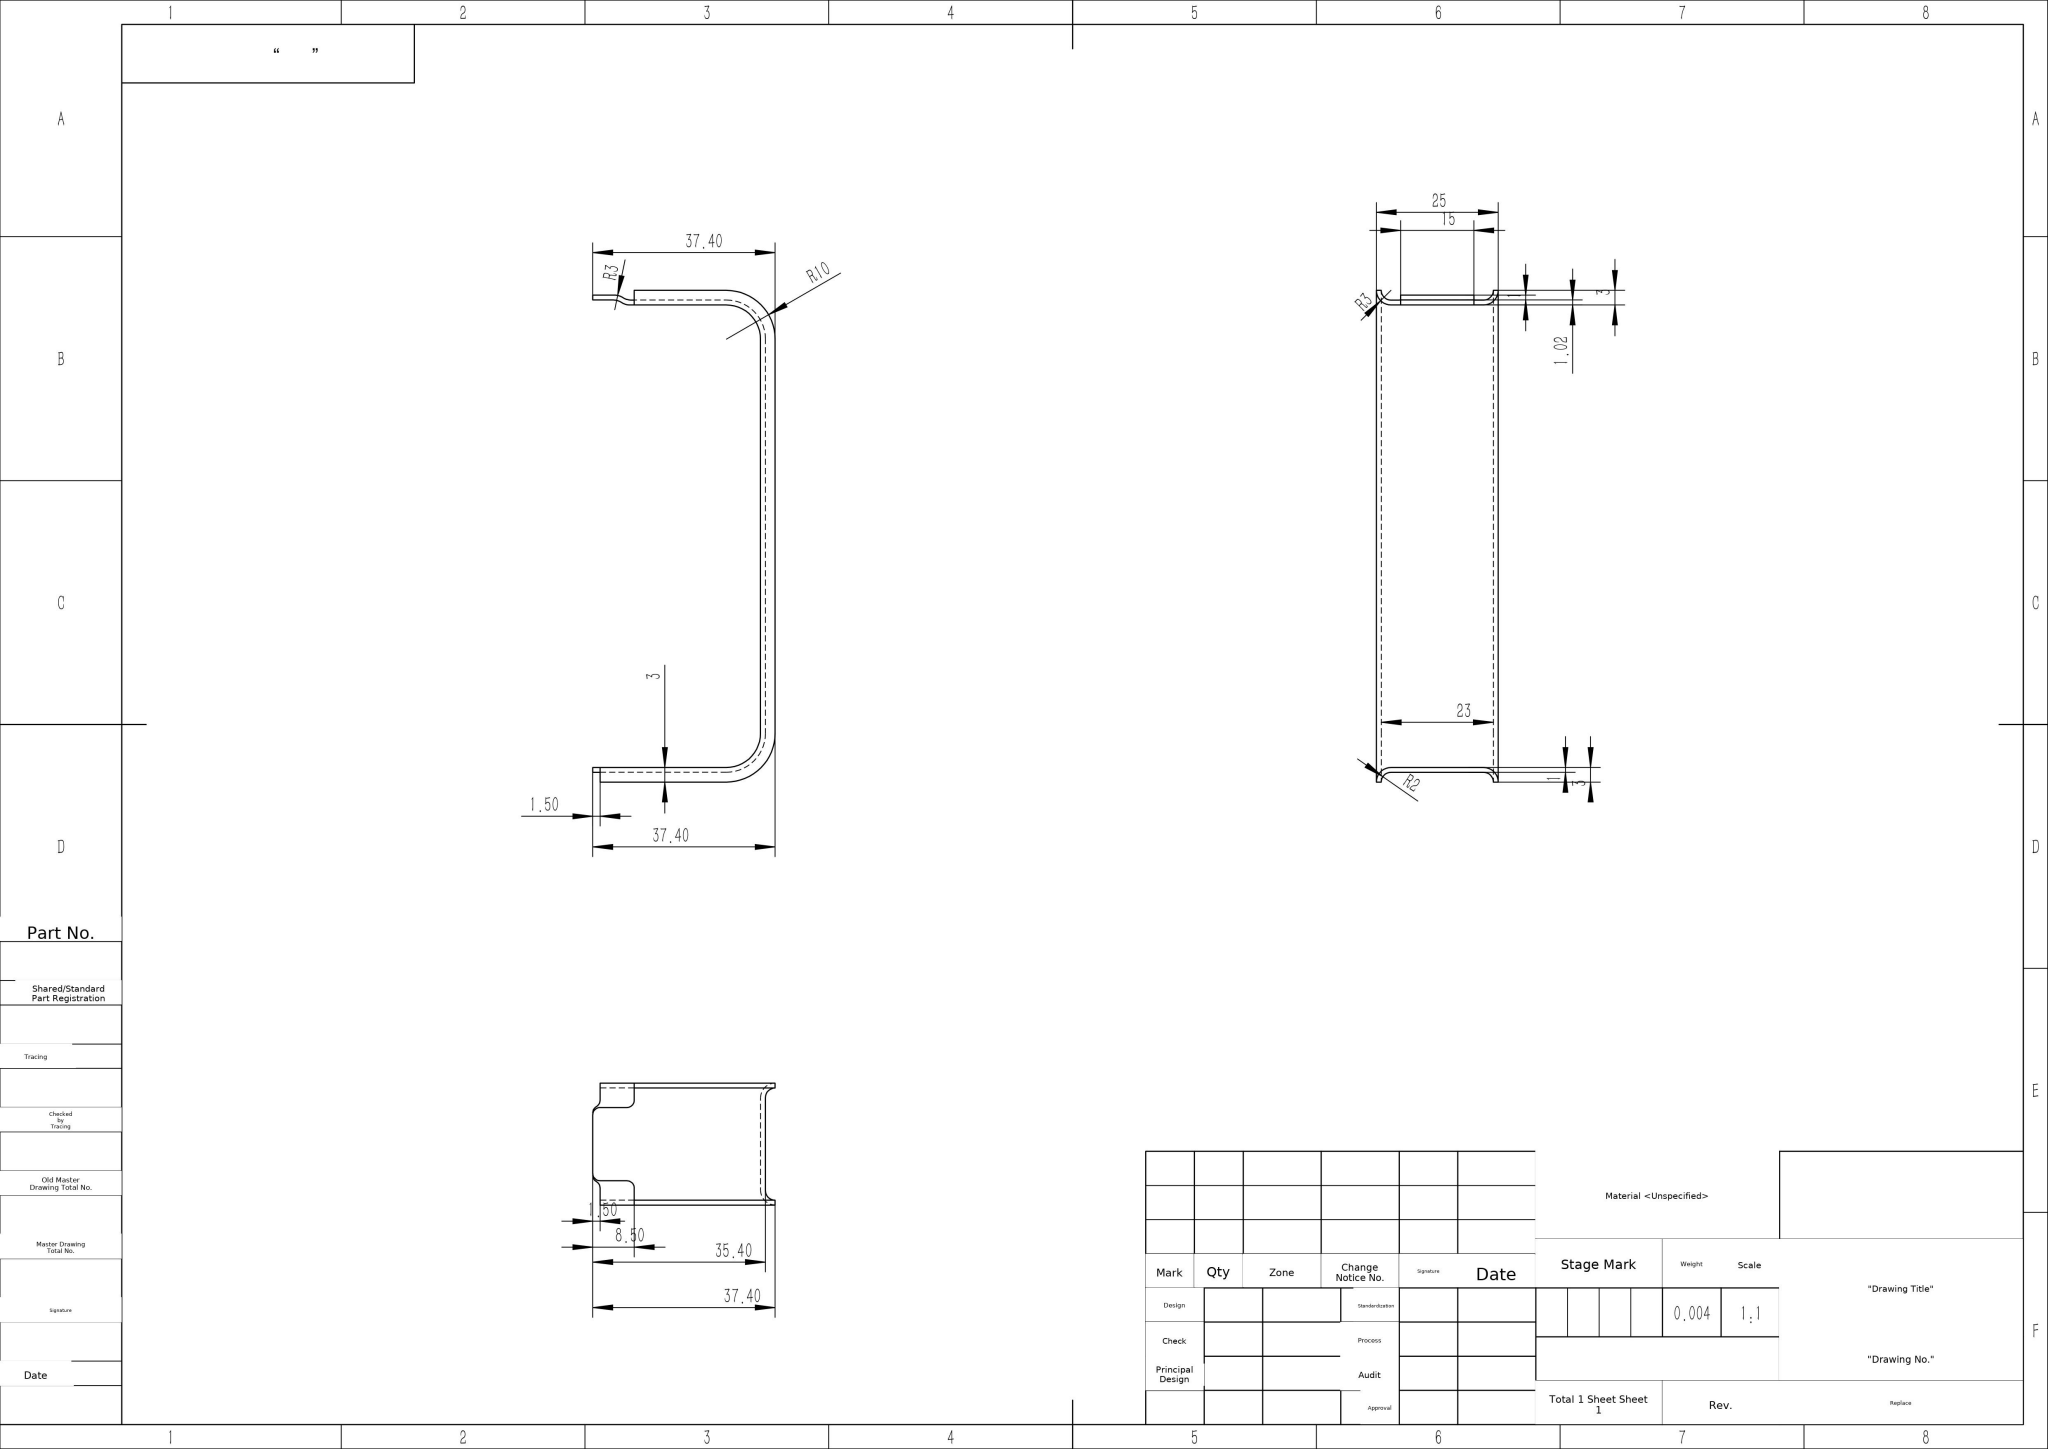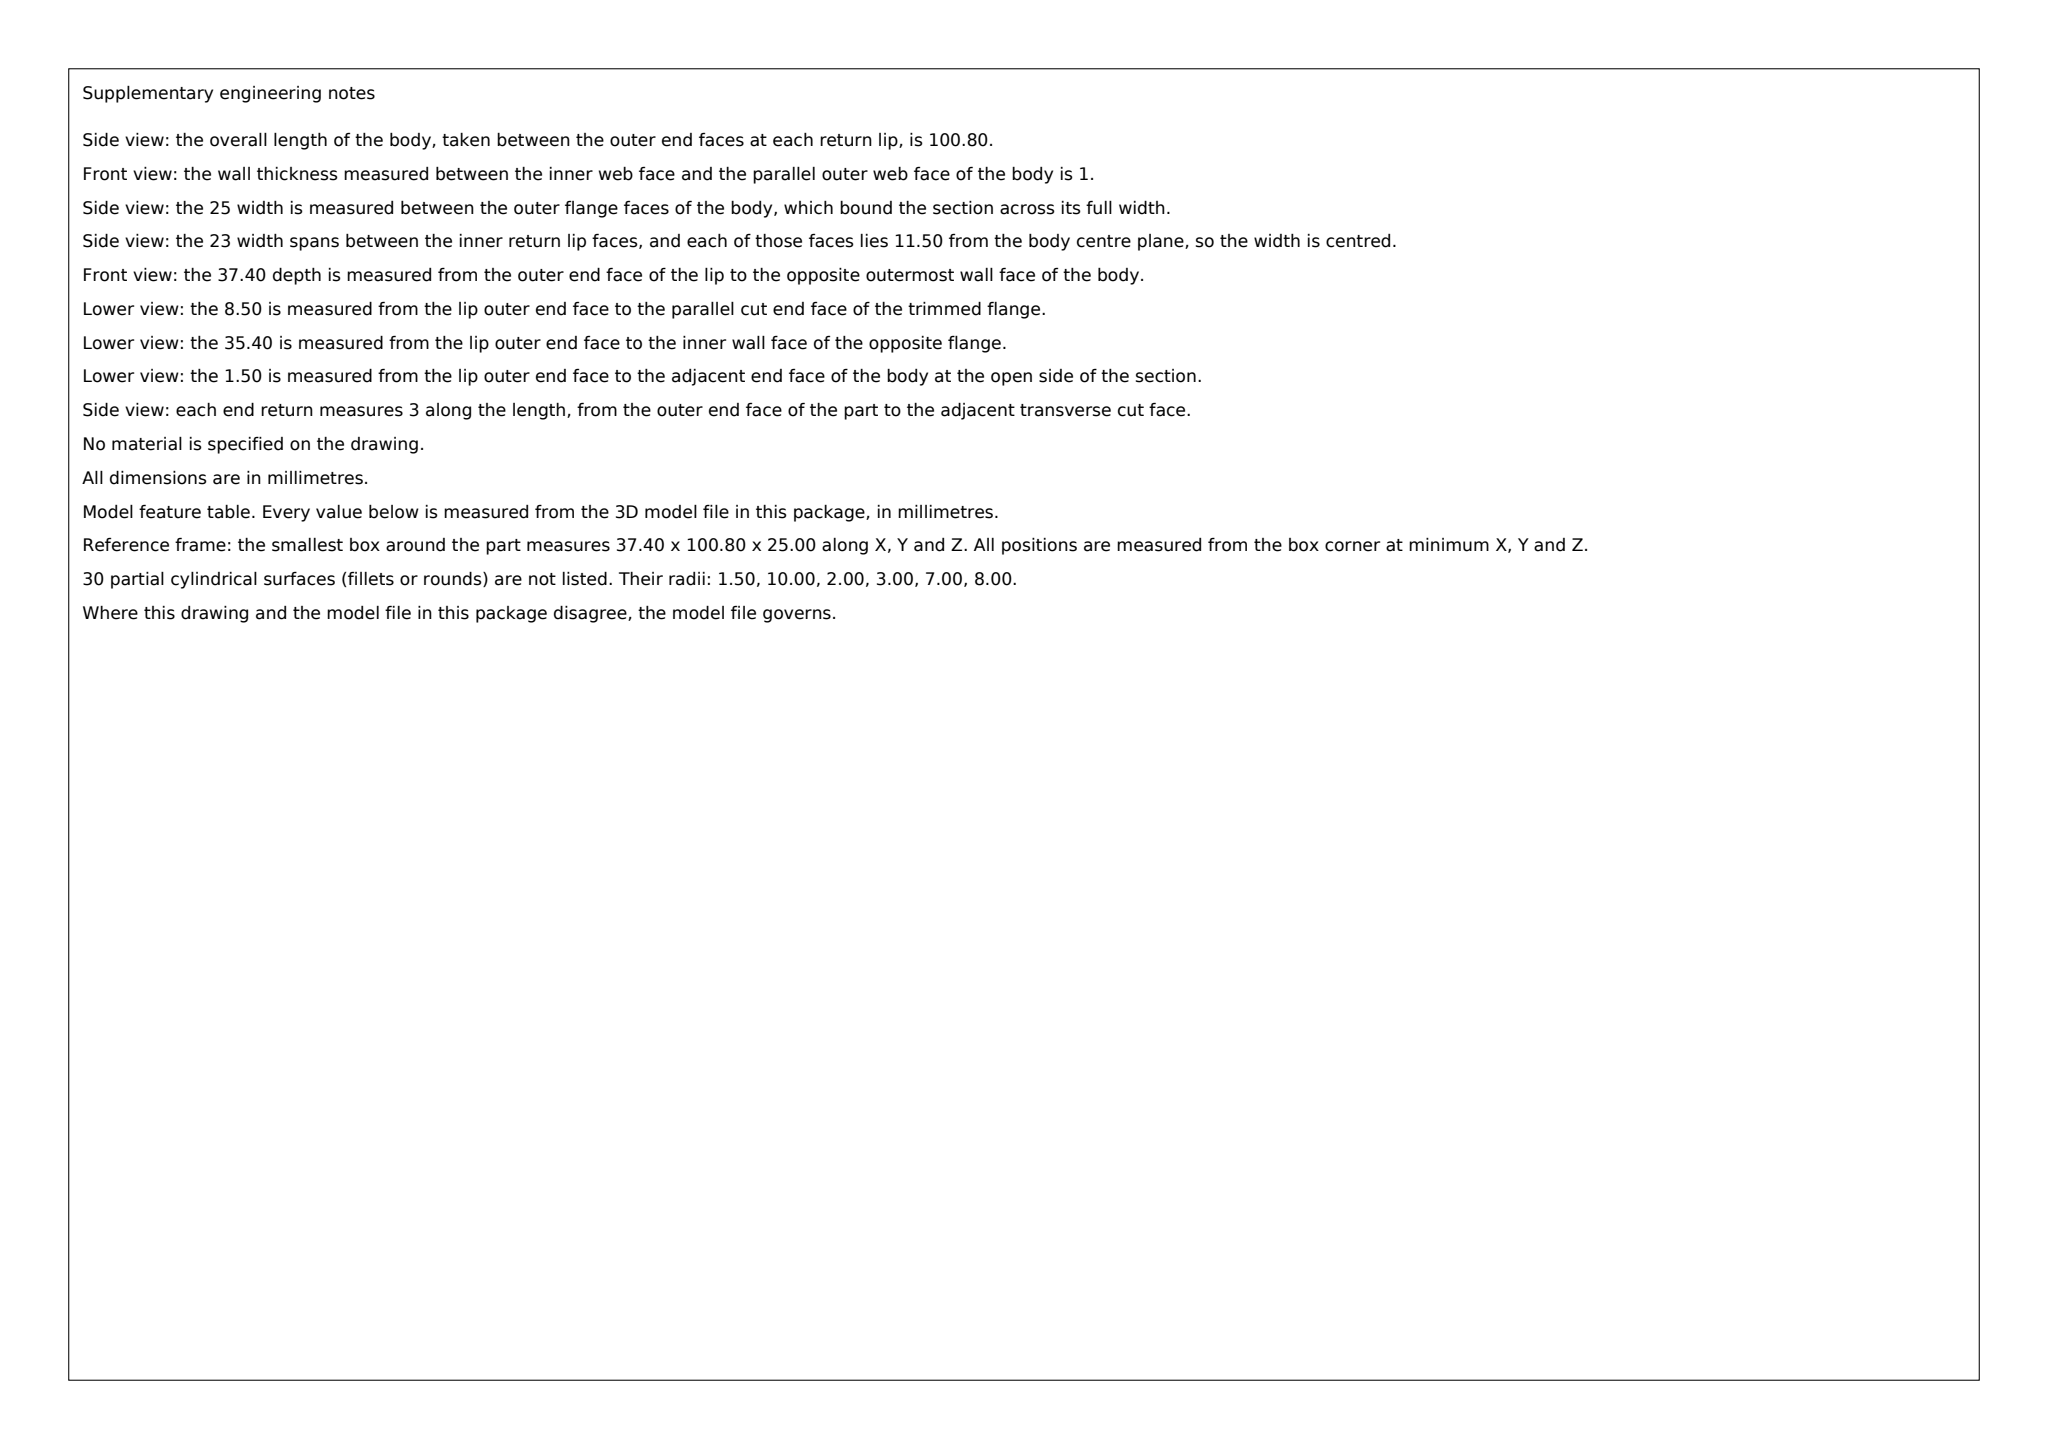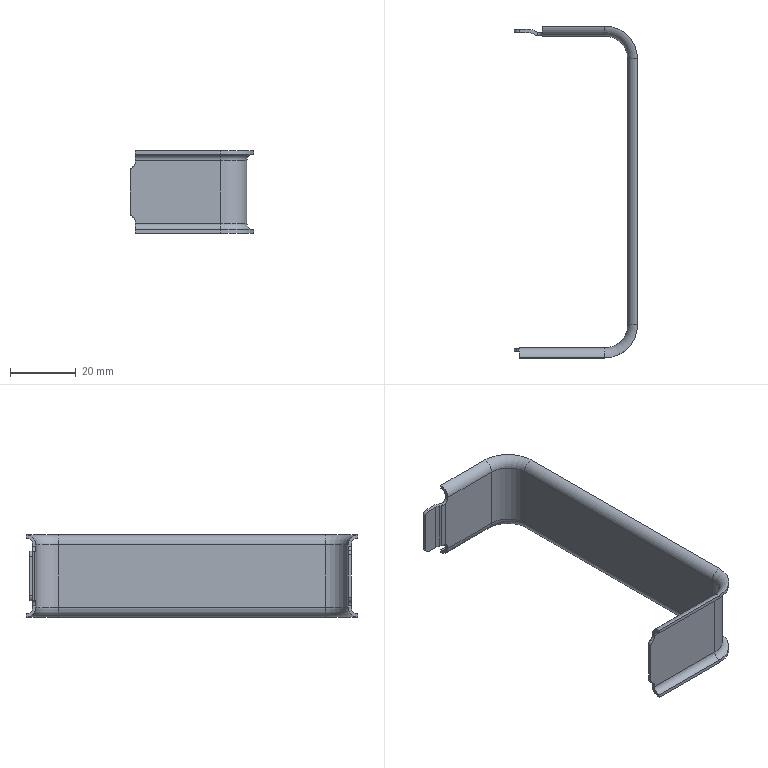Part | SolidWorks | mm | 1 solid | 64 faces | box 37.4 x 100.8 x 25 mm | volume 4182 mm3 | cylinder 32 | plane 24 | torus 8 | commonest cylinder face diameters 6 x10 3 x8 4 x6 20 x4 14 x2 16 x2
Drawing notes:
OVERALL ENVELOPE 37.40 x 107.06 x 25 | from the solid: bbox_xyz 40.529 x 107.059 x 25.0; x planes 0 to 37.4, z planes 5.0/20.0 in 25 width
SHEET THK 1.0 TYP; BEND R2 INSIDE / R3 OUTSIDE | from the solid: Coaxial bend cyls Ø4 (R2 inner) & Ø6 (R3 outer); (6-4)/2=1.0; planes x34.4/35.4 and y100.93/101.93 spaced 1.0; fillet_radii 2.0 & 3.0
BTM VIEW STEP 15 WIDE, R1.5 CNRS | from the solid: z planes 5.0 & 20.0 = 15 wide; Ø3.0 y-axis cyls (R1.5) at x0 z3.5/21.5 and x1.5 z6.1/6.5/18.5/18.9
RETURN LIP EA END 3.13 LG x 15 WIDE x 1.0 THK BEYOND 100.80 FACE | from the solid: bbox y 107.059 vs flange faces y3.13 & y103.93 (100.80 apart) = 3.13 each end; Ø6 z-axis bend cyls at (7.6,103.93)/(7.87,104.93) over 15 flat
15 WIDE RETURN LIP CTRD ON 25 WIDTH, 5 FROM EACH EDGE | from the solid: z planes at 5.0 and 20.0 within 25.0 bbox width (z 0-25): 15 wide, 5 each side
R10 OUTSIDE BEND: R8 INSIDE (TYP 2 PL) | from the solid: coaxial z-cylinders at (x27.4,y13.13) and (x27.4,y93.93): dia 20 (R10 OD) and dia 16 (R8 ID), len 19
SIDE VIEW: OAL X 40.53 = 37.40 + 3.13 R3 RETURN FLANGE PROJ | from the solid: bbox_xyz x=40.529 vs max face plane x=37.4; fillet R3; diff=3.129
BTM VIEW STEP: ENDS 5.13 & 101.93 FROM END FACE, 96.80 LG | from the solid: y planes 5.13/6.13 and 100.93/101.93 within y-extent 0 to 107.059
23 WIDE R2 FEAT SYM ABT CL OF 25 WIDTH, 1.0 EA SIDE | from the solid: z extent 25.0; x-axis cyls at z=3.0 & 22.0 and planes z=5.0/20.0 sym abt z=12.5